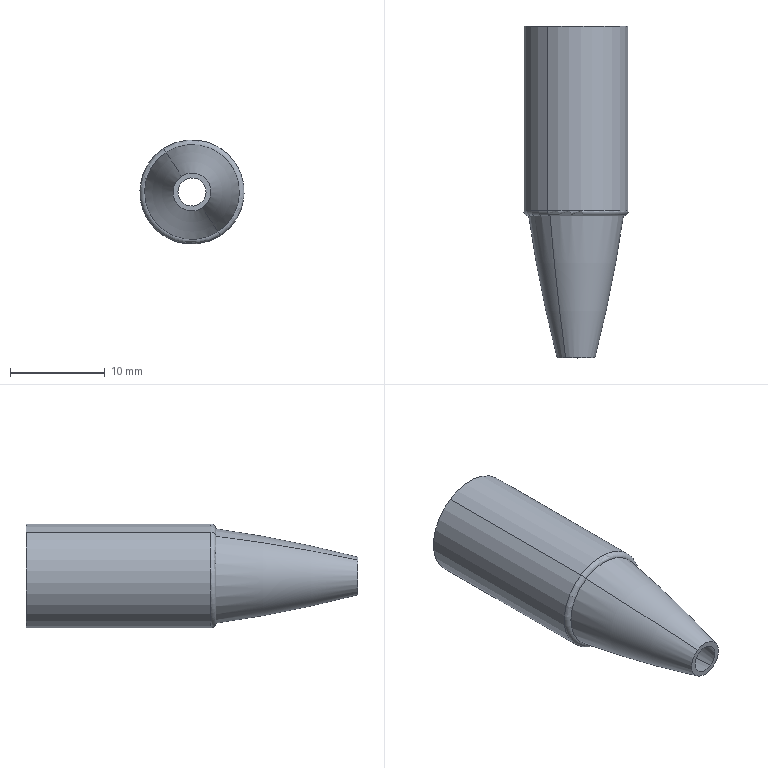Component | SolidWorks | PenTip-1 | 1 solid | 49 faces | volume 522 mm3 | cylinder 36 | torus 6 | plane 4 | spline 3 | commonest cylinder face diameters 10 x34 11 x2